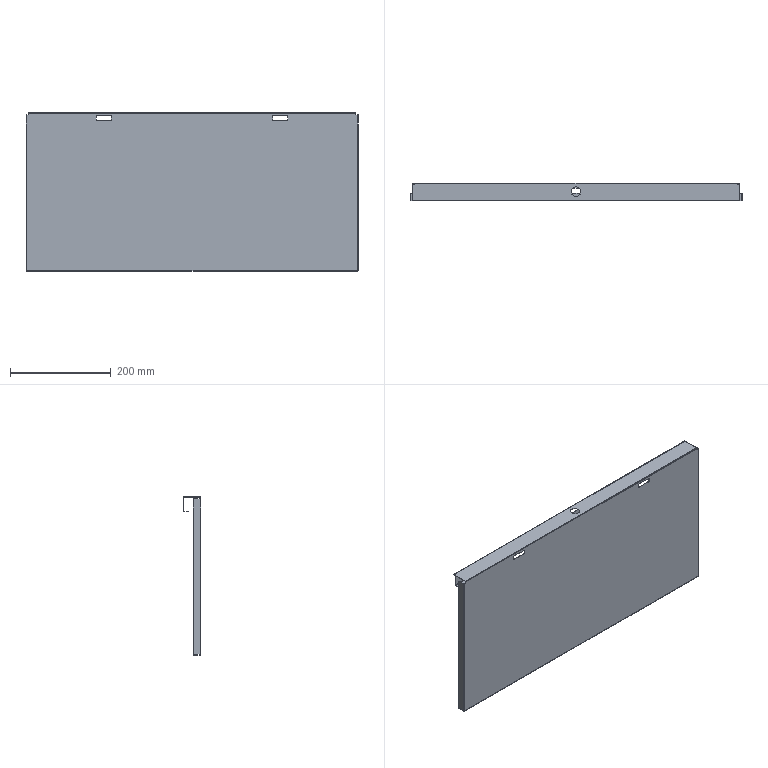Component | SolidWorks | PC-CAJ-P09-1_PM-CAJ-P38-1 | 1 solid | 90 faces | volume 186274 mm3 | plane 76 | cylinder 14 | commonest cylinder face diameters 2.4 x6 1 x6 18.708 x2 | material Plain Carbon Steel